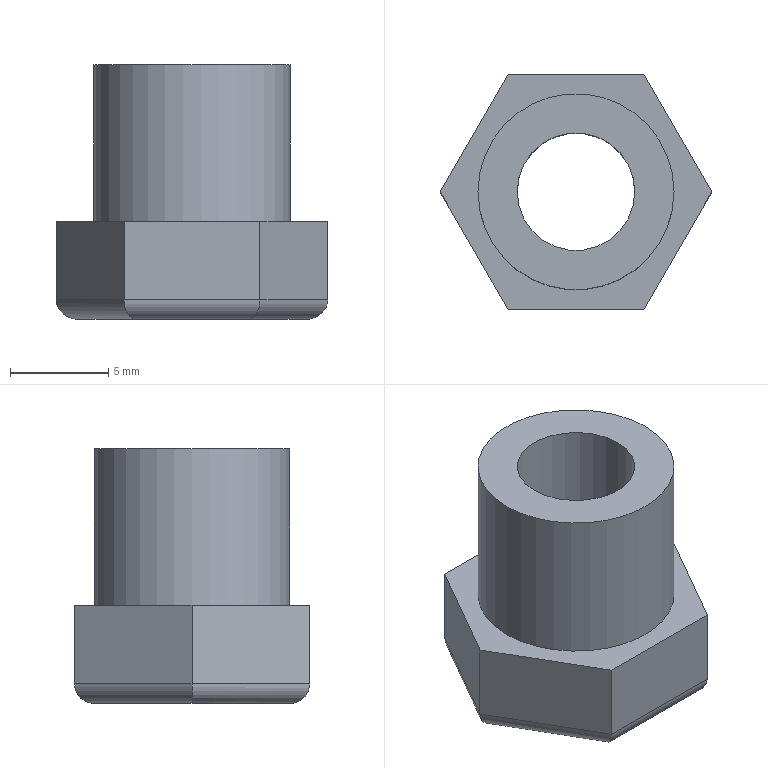Component | NX | BOTTOM_PLATE_CONNECTING_SCREW | 1 solid | 17 faces | volume 876 mm3 | plane 9 | cylinder 8 | commonest cylinder face diameters 2 x6 10 x1 6 x1